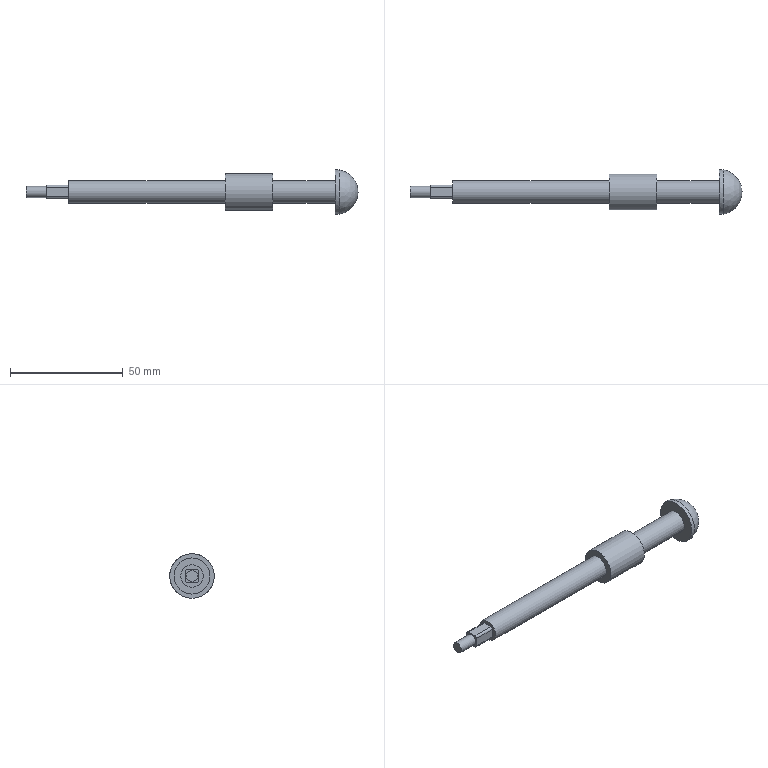Component | NX | VALVE_STEM | 1 solid | 20 faces | volume 14453 mm3 | plane 10 | cylinder 9 | sphere 1 | commonest cylinder face diameters 2 x4 10 x2 19.72 x1 16 x1 5 x1